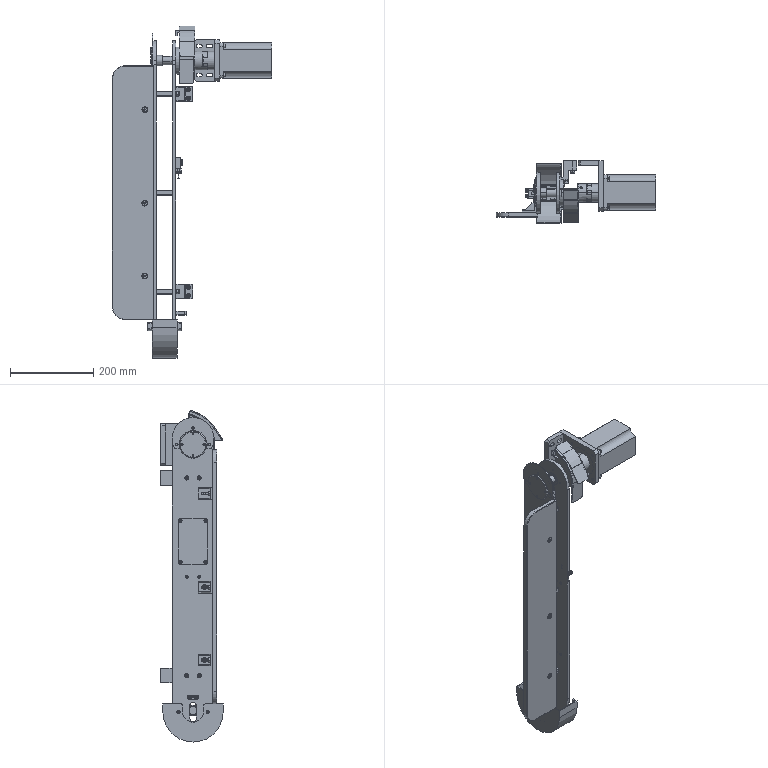Assembly | SolidWorks | mm | 101 component files | 105 solids | 2429 faces | box 382.9 x 150 x 797.7 mm | volume 3111825 mm3 | plane 1200 | cylinder 794 | cone 339 | torus 80 | sphere 12 | spline 4 | commonest cylinder face diameters 6 x114 6.68 x66 9.88 x66 5 x64 4 x49 10 x49 8.5 x32 7 x28
Bill of materials:
Deep Groove Ball Bearing, Double Sealed, 6804ZZ | 2 | 304 Stainless Steel | Flat annular ring (washer- or spacer-like): short cylinder with a large concentric through bore.
A3 Steel | 1 | A3 Steel | Thick circular flange disc with a central through bore and four small through holes evenly spaced on a bolt circle.
A3 Steel | 1 | A3 Steel | Thin circular plate with four small through holes evenly spaced on a bolt circle and no central through hole.
A3 Steel | 1 | 40Cr | Short cylindrical shaft or pin with a raised central collar and flats machined on both end sections.
A3 Steel | 2 | A3 Steel | Rectangular block with one through hole in the top face and two parallel through holes crossing it horizontally; the four vertical edges are chamfered.
Stainless Steel304 | 1 | 40Cr | Thin-walled cylindrical sleeve or bushing with chamfered edges at both ends.
A3 Steel | 1 | 40Cr | Stepped cylindrical shaft with a narrow raised ring partway along it, a reduced-diameter end journal and a keyway-like slot at the small end.
Stainless Steel304 | 1 | 40Cr | Cylindrical sleeve or bushing, longer than unnamed part, with chamfered edges at both ends.
A3 Steel | 1 | 201 Stainless Steel | Thin flat horseshoe- or C-shaped plate (partial annulus) with three small through holes: one at the crown and one near each end of the arms.
A3 Steel | 1 | A3 Steel | Long thin flat strip with fully rounded ends, a round hole at one end, an elongated slot at the other end, and several groups of very small holes along its length.
A3 Steel | 3 | A3 Steel | Rectangular block with chamfered vertical edges and two blind drilled holes on one face that end in conical drill points.
A3 Steel | 1 | A3 Steel | Rectangular flat mounting-style plate with one large circular through opening, six small through holes and two chamfered corners on one side.
A3 Steel | 1 | A3 Steel | Rectangular block-like plate with four obround through-slots in the main face, two chamfered corners on one long edge, and two small holes in one narrow side face.
A3 Steel | 1 | A3 Steel | Long, thin flat plate with rounded ends. It has a round hole near one end, an obround slot near the other end, a rectangular window toward the upper middle, and many small holes in a pattern.
A3 Steel | 1 | A3 Steel | Stepped rectangular block: a taller, narrower upper column sits on a wider, shorter base. A long obround slot passes through the column's narrow side, and the base has two round through-holes.
Stainless Steel201 | 1 | 201 Stainless Steel | Half-cylindrical, trough- or cradle-like shell with thin curved walls. One end has a flat semicircular end face with a central U-shaped cutout and two small holes, one in each flat upper tab.
A3 Steel | 2 | A3 Steel | Block with a Z-shaped, stepped profile made of two offset rectangular lobes with filleted inside corners. One face has two large through-holes; another face has three holes in a row, with the middle one smaller. The outer corners have small chamfers.
Bakelite Red | 1 | Bakelite (Red) | Long, thin flat strip with two rounded corners on one long edge and three small holes evenly spaced near the opposite edge. A small step shows at one end in the edge view.
Stainless Steel201 | 1 | 201 Stainless Steel | Bent, sheet-like bracket with a curved, angled upper flange and a flat lower tab. The flat profile has two obround slots and an irregular outline with filleted notches. A small hooked tab sticks out to one side.
Acrylic PMMA Transparent | 1 | PMMA Transparent | Thin rectangular flat plate with rounded corners and one small round hole near each of the four corners.
Coupling075-12.7-14 | 1 |  | Solid cylinder with chamfered ends and a central axial bore that appears to have a keyway. Several partial circumferential slits, offset around the circumference, cut through the body, and there is one radial hole near one end.
Foot | 3 |  | Right-angle corner bracket with two perpendicular legs joined by a solid diagonal (gusset-like) web. Each leg has one obround slot, and the leg ends have rounded corners.
GB_FASTENER_NUT_SNAB1 M6-N | 3 |  | Hexagonal nut-like prism with a plain round through-bore and chamfered corners on both faces
hex socket set screws with flat point gb | 2 |  | Short cylinder with a hexagonal socket recess in one end face and a conical, pointed or chamfered tip at the other end. There is a small chamfer at the socket end.
GB_SOCKET_TYPE7 M4X10-N | 6 |  | Pin with a domed head and a plain cylindrical shank with a flat end, like a round-head rivet or pin
GB_FASTENER_SCREWS_HSCHS M6X16-N | 3 |  | Countersunk (conical underside) flat-head fastener with a hexagonal socket recess and a plain cylindrical shank with a chamfered tip
Socket Head Cap Screw M3X20 | 2 |  | Long, slender socket-head cap-screw-like part: a cylindrical head with a hex socket and a long plain shank
GB_FASTENER_SCREWS_HSHCS M6X16-N | 16 |  | Short socket-head cap-screw-like part: a cylindrical head with a hex socket and a short, thicker plain shank
GB_FASTENER_SCREWS_HSHCS M5X25-C | 4 |  | Cylindrical-head pin or screw-like part with a long plain shank; the head's top face is not visible
GB_FASTENER_SCREWS_HSHCS M5X20-N | 4 |  | Socket-head cap-screw-like part: a cylindrical head with a hex socket and a plain cylindrical shank of medium length
GB_FASTENER_SCREWS_HSHCS M5X12-N | 2 |  | Short cylindrical-head pin or screw-like part with a thick plain shank; the head's top face is not visible
M3 Flat Washer | 2 |  | Thin flat annular washer-like disc with a central round hole
GB_FASTENER_WASHER_SMWC 6 | 2 |  | Flat annular ring/washer-like part, thicker than the thin washer, with a relatively large central hole
SlotTypeProximitySwitchEE-SX951-W | 1 |  | U-shaped, forked rectangular block with a rectangular slot between two arms. One face has two round holes, a cylindrical rod or stub sticks out from the underside, and there are small line marks on the top surface.
M4 Spring Washer | 2 |  | Split ring with a single radial cut and slightly offset ends, like a split lock washer
GB_FASTENER_WASHER_SW 6 | 14 |  | Split ring with a single radial cut and slightly offset ends, like a split lock washer; it looks nearly identical to unnamed part
M6 Spring Washer | 8 |  | Flat annular ring with a rectangular cross-section, cut through by one narrow radial split. The two cut ends look slightly offset along the axis, which fits a split (helical) lock-washer-style shape.
StepperMotor86J18118-842 | 1 |  | Elongated square-section prismatic body with concave, quarter-round reliefs running the full length of each longitudinal corner. One end has a slightly larger square flange with rounded corners and four corner through-holes, a thin raised circular boss (pilot) on its outer face, and a single plain cylindrical shaft sticking out along the central axis. The overall form looks like a compact motor-style housing with a mounting flange and output shaft.
Mates:
1. coincident | ChainPartSupport-1 face at (155.637, 19.937, -132.704) dir (1, 0, 0) | ChainPartSupport-2 face at (155.637, 19.937, -607.704) dir (1, 0, 0)
2. concentric | ChainPartInnerSidePlate-1 face at (127.637, -2.563, -35.304) dir (1, 0, 0) r 16 | ChainPartOuterSidePlate-1 face at (88.237, -2.563, -35.304) dir (-1, 0, 0) r 16
3. concentric | ChainPartInnerSidePlate-1 face at (127.637, -2.563, -670.304) dir (1, 0, 0) r 48.5 | ChainPartOuterSidePlate-1 face at (88.237, -2.563, -670.304) dir (-1, 0, 0) r 48.5
4. coincident | ChainPartInnerSidePlate-1 face at (127.637, -2.563, -35.304) dir (-1, 0, 0) | ChainPartInnerSpacer-1 face at (127.637, -2.563, -115.304) dir (1, 0, 0)
5. concentric | ChainPartInnerSidePlate-1 face at (137.637, 12.437, -115.304) dir (-1, 0, 0) r 3.5 | ChainPartInnerSpacer-1 face at (88.237, 12.437, -115.304) dir (-1, 0, 0) r 3
6. concentric | ChainPartInnerSidePlate-1 face at (137.637, -17.563, -115.304) dir (-1, 0, 0) r 3.5 | ChainPartInnerSpacer-1 face at (88.237, -17.563, -115.304) dir (-1, 0, 0) r 3
7. coincident | ChainPartOuterSidePlate-1 face at (88.237, -2.563, -35.304) dir (1, 0, 0) | ChainPartInnerSpacer-1 face at (88.237, -2.563, -115.304) dir (-1, 0, 0)
8. concentric | ChainPartInnerSidePlate-1 face at (137.637, 12.437, -590.304) dir (-1, 0, 0) r 3.5 | ChainPartInnerSpacer-3 face at (88.237, 12.437, -590.304) dir (-1, 0, 0) r 3
9. concentric | ChainPartInnerSidePlate-1 face at (127.637, -2.563, -35.304) dir (1, 0, 0) r 16 | Bearing_6804ZZ-1 face at (135.637, -2.563, -35.304) dir (-1, 0, 0) r 16
10. concentric | ChainPartDriveShaft-1 face at (198.637, -2.563, -35.304) dir (1, 0, 0) r 10 | Bearing_6804ZZ-1 face at (135.637, -2.563, -35.304) dir (-1, 0, 0) r 10
11. coincident | ChainPartDriveShaft-1 face at (128.637, -0.9828, -45.178) dir (1, 0, 0) | Bearing_6804ZZ-1 face at (128.637, 8.267, -39.461) dir (-1, 0, 0)
12. concentric | ChainPartDriveShaft-1 face at (198.637, -2.563, -35.304) dir (1, 0, 0) r 10 | Bearing_6804ZZ-2 face at (87.237, -2.563, -35.304) dir (-1, 0, 0) r 10
13. coincident | ChainPartOuterSidePlate-1 face at (80.237, -2.563, -35.304) dir (-1, 0, 0) | Bearing_6804ZZ-2 face at (80.237, 12.094, -40.931) dir (-1, 0, 0)
14. coincident | ChainPartInnerSidePlate-1 face at (135.637, -2.563, -35.304) dir (1, 0, 0) | Bearing_6804ZZ-1 face at (135.637, 11.086, -40.544) dir (1, 0, 0)
15. coincident | ChainPartInnerSidePlate-1 face at (127.637, -2.563, -35.304) dir (-1, 0, 0) | ChainPartDrivenShaft-1 face at (127.637, -15.063, -673.885) dir (1, 0, 0)
16. coincident | ChainPartInnerSidePlate-1 face at (125.637, 5.437, -662.304) dir (0, -1, 0) | ChainPartDrivenShaft-1 face at (127.637, 5.437, -693.885) dir (0, 1, 0)
17. coincident | ChainPartInnerSidePlate-1 face at (135.637, -2.563, -35.304) dir (1, 0, 0) | ChainPartBearingInnerEndCap-1 face at (135.637, 29.937, -35.304) dir (-1, 0, 0)
18. concentric | ChainPartDriveShaft-1 face at (198.637, -2.563, -35.304) dir (1, 0, 0) r 10 | ChainPartBearingInnerEndCap-1 face at (145.437, -2.563, -35.304) dir (1, 0, 0) r 10.5
19. concentric | ChainPartInnerSidePlate-1 face at (127.637, -2.563, -9.304) dir (-1, 0, 0) r 1.65 | ChainPartBearingInnerEndCap-1 face at (145.437, -2.563, -9.304) dir (1, 0, 0) r 2.25
20. coincident | ChainPartOuterSidePlate-1 face at (80.237, -2.563, -35.304) dir (-1, 0, 0) | ChainPartBearingOuterEndCap-1 face at (80.237, -35.063, -35.304) dir (1, 0, 0)
21. concentric | ChainPartOuterSidePlate-1 face at (80.737, -2.563, -35.304) dir (1, 0, 0) r 785.398 | ChainPartBearingOuterEndCap-1 face at (75.437, -2.563, -35.304) dir (-1, 0, 0) r 32.5
22. concentric | ChainPartOuterSidePlate-1 face at (88.237, 23.437, -35.304) dir (1, 0, 0) r 2 | ChainPartBearingOuterEndCap-1 face at (75.437, 23.437, -35.304) dir (-1, 0, 0) r 2.25
23. coincident | Bearing_6804ZZ-2 face at (87.237, 11.086, -40.544) dir (1, 0, 0) | ChainPartDriveShaftLocatingSleeve-1 face at (87.237, -2.563, -35.304) dir (-1, 0, 0)
24. concentric | ChainPartDriveShaft-1 face at (198.637, -2.563, -35.304) dir (1, 0, 0) r 10 | ChainPartDriveShaftLocatingSleeve-1 face at (104.337, -2.563, -35.304) dir (-1, 0, 0) r 12.5
25. coincident | ChainPartOuterSidePlate-1 face at (88.237, -2.563, -35.304) dir (1, 0, 0) | ChainPartDrivenShaftLocatingSleeve-1 face at (88.237, -2.563, -673.885) dir (-1, 0, 0)
26. concentric | ChainPartDrivenShaft-1 face at (67.237, -2.563, -673.885) dir (-1, 0, 0) r 10 | ChainPartDrivenShaftLocatingSleeve-1 face at (100.937, -2.563, -673.885) dir (-1, 0, 0) r 12.5
27. coincident | ChainPartOuterSidePlate-1 face at (80.237, -2.563, -35.304) dir (-1, 0, 0) | ChainPartWindowPlate-1 face at (80.237, -32.563, -317.804) dir (1, 0, 0)
28. concentric | ChainPartOuterSidePlate-1 face at (80.237, 27.437, -217.804) dir (-1, 0, 0) r 2 | ChainPartWindowPlate-1 face at (77.237, 27.437, -217.804) dir (1, 0, 0) r 2.25
29. concentric | ChainPartOuterSidePlate-1 face at (80.237, 27.437, -317.804) dir (-1, 0, 0) r 2 | ChainPartWindowPlate-1 face at (77.237, 27.437, -317.804) dir (1, 0, 0) r 2.25
30. concentric | ChainPartInnerSidePlate-1 face at (135.637, 4.437, -642.304) dir (1, 0, 0) r 2.5 | ChainPartDrivenShaftAdjustmentBracket-2 face at (135.637, 4.437, -642.304) dir (1, 0, 0) r 2.75
31. concentric | ChainPartInnerSidePlate-1 face at (135.637, -9.563, -642.304) dir (1, 0, 0) r 2.5 | ChainPartDrivenShaftAdjustmentBracket-2 face at (135.637, -9.563, -642.304) dir (1, 0, 0) r 2.75
32. concentric | ChainPartOuterSidePlate-1 face at (80.237, 4.437, -642.304) dir (-1, 0, 0) r 2.5 | ChainPartDrivenShaftAdjustmentBracket-4 face at (80.237, 4.437, -642.304) dir (-1, 0, 0) r 2.75
33. concentric | ChainPartOuterSidePlate-1 face at (80.237, -9.563, -642.304) dir (-1, 0, 0) r 2.5 | ChainPartDrivenShaftAdjustmentBracket-4 face at (80.237, -9.563, -642.304) dir (-1, 0, 0) r 2.75
34. concentric | ChainPartSupport-1 face at (155.637, 27.437, -125.304) dir (1, 0, 0) r 5.5 | ChainPartInnerSidePlate-1 face at (127.637, 27.437, -125.304) dir (-1, 0, 0) r 3
35. concentric | ChainPartSupport-1 face at (155.637, 27.437, -105.304) dir (1, 0, 0) r 5.5 | ChainPartInnerSidePlate-1 face at (127.637, 27.437, -105.304) dir (-1, 0, 0) r 3
36. concentric | ChainPartSupport-2 face at (155.637, 27.437, -580.304) dir (1, 0, 0) r 5.5 | ChainPartInnerSidePlate-1 face at (127.637, 27.437, -580.304) dir (-1, 0, 0) r 3
37. concentric | ChainPartSupport-2 face at (155.637, 27.437, -600.304) dir (1, 0, 0) r 5.5 | ChainPartInnerSidePlate-1 face at (127.637, 27.437, -600.304) dir (-1, 0, 0) r 3
38. concentric | ChainPartDriveShaft-1 face at (198.637, -2.563, -35.304) dir (1, 0, 0) r 7 | Coupling075-12.7-14-1 face at (199.337, -2.563, -35.304) dir (-1, 0, 0) r 7
39. coincident | ChainPartDriveShaft-1 face at (178.637, -1.457, -42.216) dir (1, 0, 0) | Coupling075-12.7-14-1 face at (178.637, -22.592, -12.658) dir (-1, 0, 0)
40. concentric | Coupling075-12.7-14-1 face at (178.636, -2.563, -35.304) dir (1, 0, 0) r 6.35 | StepperMotor86J18118-842-1 face at (209.117, -2.563, -35.304) dir (1, 0, 0) r 6.35
41. distance | StepperMotor86J18118-842-1 face at (239.117, -2.563, -35.304) dir (-1, 0, 0) | Coupling075-12.7-14-1 face at (232.737, 19.843, -15.006) dir (1, 0, 0)
42. coincident | ChainPartOuterSidePlate-1 face at (80.237, -52.063, -35.304) dir (0, -1, 0) | ChainPartTablePlate-1 face at (32.737, -52.063, -352.804) dir (0, 1, 0)
43. coincident | ChainPartOuterSidePlate-1 face at (80.237, -2.563, -35.304) dir (-1, 0, 0) | ChainPartTablePlate-1 face at (80.237, -52.063, -657.804) dir (1, 0, 0)
44. coincident | ChainPartSupport-1 face at (135.637, 74.937, -132.704) dir (-1, 0, 0) | ChainPartInnerSidePlate-1 face at (135.637, -2.563, -35.304) dir (1, 0, 0)
45. coincident | ChainPartTablePlate-1 face at (-17.263, -50.063, -657.804) dir (0, 1, 0) | Foot-1 face at (80.237, -50.063, -138.804) dir (0, -1, 0)
46. coincident | ChainPartOuterSidePlate-1 face at (80.237, -2.563, -35.304) dir (-1, 0, 0) | Foot-1 face at (80.237, -50.063, -138.804) dir (1, 0, 0)
47. coincident | ChainPartOuterSidePlate-1 face at (80.237, -2.563, -35.304) dir (-1, 0, 0) | Foot-2 face at (80.237, -50.063, -538.804) dir (1, 0, 0)
48. concentric | ChainPartOuterSidePlate-1 face at (80.237, -30.563, -552.804) dir (-1, 0, 0) r 2.5 | Foot-2 sketch point at (75.637, -30.563, -552.804) dir (1, 0, 0)
49. coincident | ChainPartOuterSidePlate-1 face at (88.237, -2.563, -35.304) dir (1, 0, 0) | ChainPartInnerSpacer-3 face at (88.237, -2.563, -590.304) dir (-1, 0, 0)
50. concentric | ChainPartBearingInnerEndCap-1 face at (145.437, -28.563, -35.304) dir (1, 0, 0) r 2.25 | ChainPartThreadGuide-1 sketch point at (160.737, -28.563, -35.304) dir (1, 0, 0)
51. coincident | ChainPartOuterSidePlate-1 face at (80.237, -2.563, -35.304) dir (-1, 0, 0) | ChainPartDrivenShaftAdjustmentBracket-4 face at (80.237, -2.563, -642.304) dir (1, 0, 0)
52. coincident | ChainPartInnerSidePlate-1 face at (135.637, -2.563, -35.304) dir (1, 0, 0) | ChainPartDrivenShaftAdjustmentBracket-2 face at (135.637, -2.563, -642.304) dir (-1, 0, 0)
53. concentric | StepperMotor86J18118-842-1 face at (365.637, -37.313, -0.5537) dir (-1, 0, 0) r 2.75 | spring lock washers--normal type gb-30 face at (249.137, -37.313, -0.5537) dir (1, 0, 0) r 3.34
54. coincident | StepperMotor86J18118-842-1 face at (249.137, -44.384, 6.517) dir (1, 0, 0) | spring lock washers--normal type gb-30 face at (249.137, -37.313, -0.5537) dir (-1, 0, 0)
55. concentric | StepperMotor86J18118-842-1 face at (365.637, -37.313, -70.054) dir (-1, 0, 0) r 2.75 | spring lock washers--normal type gb-31 face at (249.137, -37.313, -70.054) dir (1, 0, 0) r 3.34
56. coincident | StepperMotor86J18118-842-1 face at (249.137, -44.384, -77.125) dir (1, 0, 0) | spring lock washers--normal type gb-31 face at (249.137, -37.313, -70.054) dir (-1, 0, 0)
57. concentric | StepperMotor86J18118-842-1 face at (365.637, 32.187, -0.5537) dir (-1, 0, 0) r 2.75 | spring lock washers--normal type gb-28 face at (249.137, 32.187, -0.5537) dir (1, 0, 0) r 3.34
58. coincident | StepperMotor86J18118-842-1 face at (249.137, 39.258, 6.517) dir (1, 0, 0) | spring lock washers--normal type gb-28 face at (249.137, 32.187, -0.5537) dir (-1, 0, 0)
59. concentric | StepperMotor86J18118-842-1 edge at (249.137, 32.187, -70.054) dir (1, 0, 0) r 2.75 | spring lock washers--normal type gb-29 face at (249.137, 32.187, -70.054) dir (1, 0, 0) r 3.34
60. coincident | StepperMotor86J18118-842-1 face at (249.137, 39.258, -77.125) dir (1, 0, 0) | spring lock washers--normal type gb-29 face at (249.137, 32.187, -70.054) dir (-1, 0, 0)
61. concentric | StepperMotor86J18118-842-1 face at (365.637, -37.313, -0.5537) dir (-1, 0, 0) r 2.75 | hexagon socket head cap screws gb-29 face at (230.737, -37.313, -0.5537) dir (1, 0, 0) r 2.5
62. coincident | spring lock washers--normal type gb-30 face at (250.737, -37.313, -0.5537) dir (1, 0, 0) | hexagon socket head cap screws gb-29 face at (250.737, -37.313, -0.5537) dir (-1, 0, 0)
63. concentric | spring lock washers--normal type gb-31 face at (249.137, -37.313, -70.054) dir (1, 0, 0) r 3.34 | hexagon socket head cap screws gb-30 face at (230.737, -37.313, -70.054) dir (1, 0, 0) r 2.5
64. coincident | spring lock washers--normal type gb-31 face at (250.737, -37.313, -70.054) dir (1, 0, 0) | hexagon socket head cap screws gb-30 face at (250.737, -37.313, -70.054) dir (-1, 0, 0)
65. concentric | spring lock washers--normal type gb-28 face at (249.137, 32.187, -0.5537) dir (1, 0, 0) r 3.34 | hexagon socket head cap screws gb-31 face at (230.737, 32.187, -0.5537) dir (1, 0, 0) r 2.5
66. coincident | spring lock washers--normal type gb-28 face at (250.737, 32.187, -0.5537) dir (1, 0, 0) | hexagon socket head cap screws gb-31 face at (250.737, 32.187, -0.5537) dir (-1, 0, 0)
67. concentric | spring lock washers--normal type gb-29 face at (249.137, 32.187, -70.054) dir (1, 0, 0) r 3.34 | hexagon socket head cap screws gb-32 face at (230.737, 32.187, -70.054) dir (1, 0, 0) r 2.5
68. coincident | spring lock washers--normal type gb-29 face at (250.737, 32.187, -70.054) dir (1, 0, 0) | hexagon socket head cap screws gb-32 face at (250.737, 32.187, -70.054) dir (-1, 0, 0)
69. coincident | ChainPartOuterSidePlate-1 face at (80.237, -2.563, -35.304) dir (-1, 0, 0) | ChainPartRearCover-1 face at (80.237, -2.563, -677.304) dir (1, 0, 0)
70. concentric | ChainPartOuterSidePlate-1 face at (80.237, -37.563, -677.304) dir (-1, 0, 0) r 2.5 | ChainPartRearCover-1 face at (88.237, -37.563, -677.304) dir (-1, 0, 0) r 3
71. concentric | ChainPartOuterSidePlate-1 face at (80.237, 32.437, -677.304) dir (-1, 0, 0) r 2.5 | ChainPartRearCover-1 face at (88.237, 32.437, -677.304) dir (-1, 0, 0) r 3
72. concentric | ChainPartRearCover-1 face at (88.237, -37.563, -677.304) dir (-1, 0, 0) r 3 | hexagon socket button head screws gb-4 face at (88.237, -37.563, -677.304) dir (-1, 0, 0) r 2
73. coincident | ChainPartRearCover-1 face at (78.237, -2.563, -677.304) dir (-1, 0, 0) | hexagon socket button head screws gb-4 face at (78.237, -37.563, -677.304) dir (1, 0, 0)
74. concentric | ChainPartRearCover-1 face at (88.237, 32.437, -677.304) dir (-1, 0, 0) r 3 | hexagon socket button head screws gb-5 face at (88.237, 32.437, -677.304) dir (-1, 0, 0) r 2
75. coincident | ChainPartRearCover-1 face at (78.237, -2.563, -677.304) dir (-1, 0, 0) | hexagon socket button head screws gb-5 face at (78.237, 32.437, -677.304) dir (1, 0, 0)
76. concentric | ChainPartWindowPlate-1 face at (77.237, 27.437, -317.804) dir (1, 0, 0) r 2.25 | hexagon socket button head screws gb-6 face at (87.237, 27.437, -317.804) dir (-1, 0, 0) r 2
77. coincident | ChainPartWindowPlate-1 face at (77.237, -32.563, -317.804) dir (-1, 0, 0) | hexagon socket button head screws gb-6 face at (77.237, 27.437, -317.804) dir (1, 0, 0)
78. concentric | ChainPartWindowPlate-1 face at (77.237, -32.563, -317.804) dir (1, 0, 0) r 2.25 | hexagon socket button head screws gb-7 face at (87.237, -32.563, -317.804) dir (-1, 0, 0) r 2
79. coincident | ChainPartWindowPlate-1 face at (77.237, -32.563, -317.804) dir (-1, 0, 0) | hexagon socket button head screws gb-7 face at (77.237, -32.563, -317.804) dir (1, 0, 0)
80. concentric | ChainPartWindowPlate-1 face at (77.237, -32.563, -217.804) dir (1, 0, 0) r 2.25 | hexagon socket button head screws gb-8 face at (87.237, -32.563, -217.804) dir (-1, 0, 0) r 2
81. coincident | ChainPartWindowPlate-1 face at (77.237, -32.563, -317.804) dir (-1, 0, 0) | hexagon socket button head screws gb-8 face at (77.237, -32.563, -217.804) dir (1, 0, 0)
82. concentric | ChainPartWindowPlate-1 face at (77.237, 27.437, -217.804) dir (1, 0, 0) r 2.25 | hexagon socket button head screws gb-9 face at (87.237, 27.437, -217.804) dir (-1, 0, 0) r 2
83. coincident | ChainPartWindowPlate-1 face at (77.237, -32.563, -317.804) dir (-1, 0, 0) | hexagon socket button head screws gb-9 face at (77.237, 27.437, -217.804) dir (1, 0, 0)
84. concentric | ChainPartInnerSidePlate-1 face at (137.637, -17.563, -590.304) dir (-1, 0, 0) r 3.5 | ChainPartInnerSpacer-3 face at (88.237, -17.563, -590.304) dir (-1, 0, 0) r 3
85. concentric | ChainPartOuterSidePlate-1 face at (78.237, -17.563, -115.304) dir (1, 0, 0) r 3.5 | spring lock washers--normal type gb-16 face at (80.237, -17.563, -115.304) dir (-1, 0, 0) r 3.34
86. coincident | ChainPartOuterSidePlate-1 face at (80.237, -2.563, -35.304) dir (-1, 0, 0) | spring lock washers--normal type gb-16 face at (80.237, -17.563, -115.304) dir (1, 0, 0)
87. concentric | ChainPartOuterSidePlate-1 face at (78.237, 12.437, -115.304) dir (1, 0, 0) r 3.5 | spring lock washers--normal type gb-17 face at (80.237, 12.437, -115.304) dir (-1, 0, 0) r 3.34
88. coincident | ChainPartOuterSidePlate-1 face at (80.237, -2.563, -35.304) dir (-1, 0, 0) | spring lock washers--normal type gb-17 face at (80.237, 12.437, -115.304) dir (1, 0, 0)
89. concentric | ChainPartOuterSidePlate-1 face at (78.237, -17.563, -590.304) dir (1, 0, 0) r 3.5 | spring lock washers--normal type gb-18 face at (80.237, -17.563, -590.304) dir (-1, 0, 0) r 3.34
90. coincident | ChainPartOuterSidePlate-1 face at (80.237, -2.563, -35.304) dir (-1, 0, 0) | spring lock washers--normal type gb-18 face at (80.237, -17.563, -590.304) dir (1, 0, 0)
91. concentric | ChainPartOuterSidePlate-1 face at (78.237, 12.437, -590.304) dir (1, 0, 0) r 3.5 | spring lock washers--normal type gb-19 face at (80.237, 12.437, -590.304) dir (-1, 0, 0) r 3.34
92. coincident | ChainPartOuterSidePlate-1 face at (80.237, -2.563, -35.304) dir (-1, 0, 0) | spring lock washers--normal type gb-19 face at (80.237, 12.437, -590.304) dir (1, 0, 0)
93. concentric | ChainPartInnerSidePlate-1 face at (137.637, -17.563, -115.304) dir (-1, 0, 0) r 3.5 | spring lock washers--normal type gb-20 face at (135.637, -17.563, -115.304) dir (1, 0, 0) r 3.34
94. coincident | ChainPartInnerSidePlate-1 face at (135.637, -2.563, -35.304) dir (1, 0, 0) | spring lock washers--normal type gb-20 face at (135.637, -17.563, -115.304) dir (-1, 0, 0)
95. concentric | ChainPartInnerSidePlate-1 face at (137.637, 12.437, -115.304) dir (-1, 0, 0) r 3.5 | spring lock washers--normal type gb-21 face at (135.637, 12.437, -115.304) dir (1, 0, 0) r 3.34
96. coincident | ChainPartInnerSidePlate-1 face at (135.637, -2.563, -35.304) dir (1, 0, 0) | spring lock washers--normal type gb-21 face at (135.637, 12.437, -115.304) dir (-1, 0, 0)
97. concentric | ChainPartInnerSidePlate-1 face at (137.637, -17.563, -590.304) dir (-1, 0, 0) r 3.5 | spring lock washers--normal type gb-22 face at (135.637, -17.563, -590.304) dir (1, 0, 0) r 3.34
98. coincident | ChainPartInnerSidePlate-1 face at (135.637, -2.563, -35.304) dir (1, 0, 0) | spring lock washers--normal type gb-22 face at (135.637, -17.563, -590.304) dir (-1, 0, 0)
99. concentric | ChainPartInnerSidePlate-1 face at (137.637, 12.437, -590.304) dir (-1, 0, 0) r 3.5 | spring lock washers--normal type gb-23 face at (135.637, 12.437, -590.304) dir (1, 0, 0) r 3.34
100. coincident | ChainPartInnerSidePlate-1 face at (135.637, -2.563, -35.304) dir (1, 0, 0) | spring lock washers--normal type gb-23 face at (135.637, 12.437, -590.304) dir (-1, 0, 0)
101. concentric | spring lock washers--normal type gb-19 face at (80.237, 12.437, -590.304) dir (-1, 0, 0) r 4.94 | hexagon socket head cap screws gb-17 face at (94.637, 12.437, -590.304) dir (-1, 0, 0) r 3
102. coincident | spring lock washers--normal type gb-19 face at (78.637, 12.437, -590.304) dir (-1, 0, 0) | hexagon socket head cap screws gb-17 face at (78.637, 12.437, -590.304) dir (1, 0, 0)
103. concentric | spring lock washers--normal type gb-18 face at (80.237, -17.563, -590.304) dir (-1, 0, 0) r 3.34 | hexagon socket head cap screws gb-18 face at (94.637, -17.563, -590.304) dir (-1, 0, 0) r 3
104. coincident | spring lock washers--normal type gb-18 face at (78.637, -17.563, -590.304) dir (-1, 0, 0) | hexagon socket head cap screws gb-18 face at (78.637, -17.563, -590.304) dir (1, 0, 0)
105. concentric | spring lock washers--normal type gb-16 face at (80.237, -17.563, -115.304) dir (-1, 0, 0) r 3.34 | hexagon socket head cap screws gb-19 face at (94.637, -17.563, -115.304) dir (-1, 0, 0) r 3
106. coincident | spring lock washers--normal type gb-16 face at (78.637, -17.563, -115.304) dir (-1, 0, 0) | hexagon socket head cap screws gb-19 face at (78.637, -17.563, -115.304) dir (1, 0, 0)
107. concentric | spring lock washers--normal type gb-17 face at (80.237, 12.437, -115.304) dir (-1, 0, 0) r 3.34 | hexagon socket head cap screws gb-20 face at (94.637, 12.437, -115.304) dir (-1, 0, 0) r 3
108. coincident | spring lock washers--normal type gb-17 face at (78.637, 12.437, -115.304) dir (-1, 0, 0) | hexagon socket head cap screws gb-20 face at (78.637, 12.437, -115.304) dir (1, 0, 0)
109. concentric | spring lock washers--normal type gb-20 face at (135.637, -17.563, -115.304) dir (1, 0, 0) r 3.34 | hexagon socket head cap screws gb-21 face at (121.237, -17.563, -115.304) dir (1, 0, 0) r 3
110. coincident | spring lock washers--normal type gb-20 face at (137.237, -17.563, -115.304) dir (1, 0, 0) | hexagon socket head cap screws gb-21 face at (137.237, -17.563, -115.304) dir (-1, 0, 0)
111. concentric | spring lock washers--normal type gb-21 face at (135.637, 12.437, -115.304) dir (1, 0, 0) r 3.34 | hexagon socket head cap screws gb-22 face at (121.237, 12.437, -115.304) dir (1, 0, 0) r 3
112. coincident | spring lock washers--normal type gb-21 face at (137.237, 12.437, -115.304) dir (1, 0, 0) | hexagon socket head cap screws gb-22 face at (137.237, 12.437, -115.304) dir (-1, 0, 0)
113. concentric | spring lock washers--normal type gb-22 face at (135.637, -17.563, -590.304) dir (1, 0, 0) r 3.34 | hexagon socket head cap screws gb-23 face at (121.237, -17.563, -590.304) dir (1, 0, 0) r 3
114. coincident | spring lock washers--normal type gb-22 face at (137.237, -17.563, -590.304) dir (1, 0, 0) | hexagon socket head cap screws gb-23 face at (137.237, -17.563, -590.304) dir (-1, 0, 0)
115. concentric | spring lock washers--normal type gb-23 face at (135.637, 12.437, -590.304) dir (1, 0, 0) r 3.34 | hexagon socket head cap screws gb-24 face at (121.237, 12.437, -590.304) dir (1, 0, 0) r 3
116. coincident | spring lock washers--normal type gb-23 face at (137.237, 12.437, -590.304) dir (1, 0, 0) | hexagon socket head cap screws gb-24 face at (137.237, 12.437, -590.304) dir (-1, 0, 0)
117. concentric | ChainPartDrivenShaftAdjustmentBracket-4 face at (80.237, -9.563, -642.304) dir (-1, 0, 0) r 2.75 | spring lock washers--normal type gb-24 face at (60.437, -9.563, -642.304) dir (-1, 0, 0) r 3.34
118. coincident | ChainPartDrivenShaftAdjustmentBracket-4 face at (60.437, -2.563, -642.304) dir (-1, 0, 0) | spring lock washers--normal type gb-24 face at (60.437, -9.563, -642.304) dir (1, 0, 0)
119. concentric | ChainPartDrivenShaftAdjustmentBracket-4 face at (80.237, 4.437, -642.304) dir (-1, 0, 0) r 2.75 | spring lock washers--normal type gb-25 face at (60.437, 4.437, -642.304) dir (-1, 0, 0) r 3.34
120. coincident | ChainPartDrivenShaftAdjustmentBracket-4 face at (60.437, -2.563, -642.304) dir (-1, 0, 0) | spring lock washers--normal type gb-25 face at (60.437, 4.437, -642.304) dir (1, 0, 0)
121. concentric | ChainPartDrivenShaftAdjustmentBracket-2 face at (135.637, -9.563, -642.304) dir (1, 0, 0) r 2.75 | spring lock washers--normal type gb-26 face at (155.437, -9.563, -642.304) dir (1, 0, 0) r 3.34
122. coincident | ChainPartDrivenShaftAdjustmentBracket-2 face at (155.437, -2.563, -642.304) dir (1, 0, 0) | spring lock washers--normal type gb-26 face at (155.437, -9.563, -642.304) dir (-1, 0, 0)
123. concentric | ChainPartDrivenShaftAdjustmentBracket-2 face at (135.637, 4.437, -642.304) dir (1, 0, 0) r 2.75 | spring lock washers--normal type gb-27 face at (155.437, 4.437, -642.304) dir (1, 0, 0) r 3.34
124. coincident | ChainPartDrivenShaftAdjustmentBracket-2 face at (155.437, -2.563, -642.304) dir (1, 0, 0) | spring lock washers--normal type gb-27 face at (155.437, 4.437, -642.304) dir (-1, 0, 0)
125. concentric | ChainPartDrivenShaftAdjustmentBracket-4 face at (80.237, -9.563, -642.304) dir (-1, 0, 0) r 2.75 | hexagon socket head cap screws gb-25 face at (83.837, -9.563, -642.304) dir (-1, 0, 0) r 2.5
126. coincident | spring lock washers--normal type gb-24 face at (58.837, -9.563, -642.304) dir (-1, 0, 0) | hexagon socket head cap screws gb-25 face at (58.837, -9.563, -642.304) dir (1, 0, 0)
127. concentric | spring lock washers--normal type gb-25 face at (60.437, 4.437, -642.304) dir (-1, 0, 0) r 3.34 | hexagon socket head cap screws gb-26 face at (83.837, 4.437, -642.304) dir (-1, 0, 0) r 2.5
128. coincident | spring lock washers--normal type gb-25 face at (58.837, 4.437, -642.304) dir (-1, 0, 0) | hexagon socket head cap screws gb-26 face at (58.837, 4.437, -642.304) dir (1, 0, 0)
129. concentric | spring lock washers--normal type gb-26 face at (155.437, -9.563, -642.304) dir (1, 0, 0) r 3.34 | hexagon socket head cap screws gb-27 face at (132.037, -9.563, -642.304) dir (1, 0, 0) r 2.5
130. coincident | spring lock washers--normal type gb-26 face at (157.037, -9.563, -642.304) dir (1, 0, 0) | hexagon socket head cap screws gb-27 face at (157.037, -9.563, -642.304) dir (-1, 0, 0)
131. concentric | spring lock washers--normal type gb-27 face at (155.437, 4.437, -642.304) dir (1, 0, 0) r 3.34 | hexagon socket head cap screws gb-28 face at (132.037, 4.437, -642.304) dir (1, 0, 0) r 2.5
132. coincident | spring lock washers--normal type gb-27 face at (157.037, 4.437, -642.304) dir (1, 0, 0) | hexagon socket head cap screws gb-28 face at (157.037, 4.437, -642.304) dir (-1, 0, 0)
133. concentric | ChainPartSupport-2 face at (155.637, 27.437, -580.304) dir (1, 0, 0) r 3.25 | hexagon socket head cap screws gb-9 face at (132.637, 27.437, -580.304) dir (1, 0, 0) r 3
134. coincident | ChainPartSupport-2 face at (148.637, 24.187, -580.304) dir (1, 0, 0) | hexagon socket head cap screws gb-9 face at (148.637, 27.437, -580.304) dir (-1, 0, 0)
135. concentric | ChainPartSupport-2 face at (155.637, 27.437, -600.304) dir (1, 0, 0) r 5.5 | hexagon socket head cap screws gb-10 face at (132.637, 27.437, -600.304) dir (1, 0, 0) r 3
136. coincident | ChainPartSupport-2 face at (148.637, 24.187, -600.304) dir (1, 0, 0) | hexagon socket head cap screws gb-10 face at (148.637, 27.437, -600.304) dir (-1, 0, 0)
137. concentric | ChainPartSupport-1 face at (155.637, 27.437, -105.304) dir (1, 0, 0) r 5.5 | hexagon socket head cap screws gb-11 face at (132.637, 27.437, -105.304) dir (1, 0, 0) r 3
138. coincident | ChainPartSupport-1 face at (148.637, 24.187, -105.304) dir (1, 0, 0) | hexagon socket head cap screws gb-11 face at (148.637, 27.437, -105.304) dir (-1, 0, 0)
139. concentric | ChainPartSupport-1 face at (155.637, 27.437, -125.304) dir (1, 0, 0) r 5.5 | hexagon socket head cap screws gb-12 face at (132.637, 27.437, -125.304) dir (1, 0, 0) r 3
140. coincident | ChainPartSupport-1 face at (148.637, 24.187, -125.304) dir (1, 0, 0) | hexagon socket head cap screws gb-12 face at (148.637, 27.437, -125.304) dir (-1, 0, 0)
141. concentric | ChainPartSupport-2 face at (165.637, 51.937, -580.304) dir (0, -1, 0) r 4.5 | spring lock washers--normal type gb-12 face at (165.637, 51.937, -580.304) dir (0, -1, 0) r 3.34
142. coincident | ChainPartSupport-2 face at (155.637, 51.937, -607.704) dir (0, -1, 0) | spring lock washers--normal type gb-12 face at (165.637, 51.937, -580.304) dir (0, 1, 0)
143. concentric | ChainPartSupport-2 face at (165.637, 51.937, -600.304) dir (0, -1, 0) r 4.5 | spring lock washers--normal type gb-13 face at (165.637, 51.937, -600.304) dir (0, -1, 0) r 3.34
144. coincident | ChainPartSupport-2 face at (155.637, 51.937, -607.704) dir (0, -1, 0) | spring lock washers--normal type gb-13 face at (165.637, 51.937, -600.304) dir (0, 1, 0)
145. concentric | ChainPartSupport-1 face at (165.637, 51.937, -125.304) dir (0, -1, 0) r 4.5 | spring lock washers--normal type gb-14 face at (165.637, 51.937, -125.304) dir (0, -1, 0) r 3.34
146. coincident | ChainPartSupport-1 face at (155.637, 51.937, -132.704) dir (0, -1, 0) | spring lock washers--normal type gb-14 face at (165.637, 51.937, -125.304) dir (0, 1, 0)
147. concentric | ChainPartSupport-1 face at (165.637, 51.937, -105.304) dir (0, -1, 0) r 4.5 | spring lock washers--normal type gb-15 face at (165.637, 51.937, -105.304) dir (0, -1, 0) r 3.34
148. coincident | ChainPartSupport-1 edge at (165.637, 51.937, -105.304) dir (0, -1, 0) r 4.5 | spring lock washers--normal type gb-15 face at (165.637, 51.937, -105.304) dir (0, 1, 0)
149. concentric | ChainPartSupport-2 face at (165.637, 51.937, -600.304) dir (0, -1, 0) r 4.5 | hexagon socket head cap screws gb-13 face at (165.637, 66.337, -600.304) dir (0, -1, 0) r 3
150. coincident | spring lock washers--normal type gb-13 face at (165.637, 50.337, -600.304) dir (0, -1, 0) | hexagon socket head cap screws gb-13 face at (165.637, 50.337, -600.304) dir (0, 1, 0)
151. concentric | spring lock washers--normal type gb-12 face at (165.637, 51.937, -580.304) dir (0, -1, 0) r 3.34 | hexagon socket head cap screws gb-14 face at (165.637, 66.337, -580.304) dir (0, -1, 0) r 3
152. coincident | spring lock washers--normal type gb-12 face at (165.637, 50.337, -580.304) dir (0, -1, 0) | hexagon socket head cap screws gb-14 face at (165.637, 50.337, -580.304) dir (0, 1, 0)
153. concentric | spring lock washers--normal type gb-14 face at (165.637, 51.937, -125.304) dir (0, -1, 0) r 3.34 | hexagon socket head cap screws gb-15 face at (165.637, 66.337, -125.304) dir (0, -1, 0) r 3
154. coincident | spring lock washers--normal type gb-14 face at (165.637, 50.337, -125.304) dir (0, -1, 0) | hexagon socket head cap screws gb-15 face at (165.637, 50.337, -125.304) dir (0, 1, 0)
155. concentric | spring lock washers--normal type gb-15 face at (165.637, 51.937, -105.304) dir (0, -1, 0) r 3.34 | hexagon socket head cap screws gb-16 face at (165.637, 66.337, -105.304) dir (0, -1, 0) r 3
156. coincident | spring lock washers--normal type gb-15 face at (165.637, 50.337, -105.304) dir (0, -1, 0) | hexagon socket head cap screws gb-16 face at (165.637, 50.337, -105.304) dir (0, 1, 0)
157. concentric | ChainPartInnerSidePlate-1 face at (135.637, -33.063, -275.554) dir (1, 0, 0) r 1.5 | plain washers--product grade c gb-3 face at (147.737, -33.063, -275.554) dir (1, 0, 0) r 1.6
158. concentric | ChainPartInnerSidePlate-1 face at (135.637, -33.063, -283.554) dir (1, 0, 0) r 1.5 | plain washers--product grade c gb-4 face at (147.737, -33.063, -283.554) dir (1, 0, 0) r 1.6
159. concentric | plain washers--product grade c gb-3 face at (147.737, -33.063, -275.554) dir (1, 0, 0) r 1.6 | spring lock washers--normal type gb-1 face at (148.237, -33.063, -275.554) dir (1, 0, 0) r 2.2
160. coincident | plain washers--product grade c gb-3 face at (148.237, -33.063, -275.554) dir (1, 0, 0) | spring lock washers--normal type gb-1 face at (148.237, -33.063, -275.554) dir (-1, 0, 0)
161. concentric | plain washers--product grade c gb-4 face at (147.737, -33.063, -283.554) dir (1, 0, 0) r 1.6 | spring lock washers--normal type gb-2 face at (148.237, -33.063, -283.554) dir (1, 0, 0) r 2.2
162. coincident | plain washers--product grade c gb-4 face at (148.237, -33.063, -283.554) dir (1, 0, 0) | spring lock washers--normal type gb-2 face at (148.237, -33.063, -283.554) dir (-1, 0, 0)
163. concentric | spring lock washers--normal type gb-2 face at (148.237, -33.063, -283.554) dir (1, 0, 0) r 2.2 | hexagon socket head cap screws gb-1 face at (129.337, -33.063, -283.554) dir (1, 0, 0) r 1.5
164. coincident | spring lock washers--normal type gb-2 face at (149.337, -33.063, -283.554) dir (1, 0, 0) | hexagon socket head cap screws gb-1 face at (149.337, -33.063, -283.554) dir (-1, 0, 0)
165. concentric | spring lock washers--normal type gb-1 face at (148.237, -33.063, -275.554) dir (1, 0, 0) r 2.2 | hexagon socket head cap screws gb-2 face at (129.337, -33.063, -275.554) dir (1, 0, 0) r 1.5
166. coincident | spring lock washers--normal type gb-1 face at (149.337, -33.063, -275.554) dir (1, 0, 0) | hexagon socket head cap screws gb-2 face at (149.337, -33.063, -275.554) dir (-1, 0, 0)
167. concentric | ChainPartOuterSidePlate-1 face at (80.237, -30.563, -377.804) dir (-1, 0, 0) r 2.5 | plain washers--product grade c gb-5 face at (74.037, -30.563, -377.804) dir (1, 0, 0) r 3.3
168. concentric | ChainPartOuterSidePlate-1 face at (80.237, -30.563, -552.804) dir (-1, 0, 0) r 2.5 | plain washers--product grade c gb-6 face at (74.037, -30.563, -552.804) dir (1, 0, 0) r 3.3
169. parallel | ChainPartTablePlate-1 face at (-17.263, -50.063, -657.804) dir (0, 1, 0) | Foot-2 face at (75.637, -45.463, -538.804) dir (0, 1, 0)
170. concentric | plain washers--product grade c gb-5 face at (74.037, -30.563, -377.804) dir (1, 0, 0) r 3.3 | spring lock washers--normal type gb-10 face at (74.037, -30.563, -377.804) dir (-1, 0, 0) r 3.34
171. coincident | plain washers--product grade c gb-5 face at (74.037, -30.563, -377.804) dir (-1, 0, 0) | spring lock washers--normal type gb-10 face at (74.037, -30.563, -377.804) dir (1, 0, 0)
172. concentric | plain washers--product grade c gb-6 face at (74.037, -30.563, -552.804) dir (1, 0, 0) r 3.3 | spring lock washers--normal type gb-11 face at (74.037, -30.563, -552.804) dir (-1, 0, 0) r 3.34
173. coincident | plain washers--product grade c gb-6 face at (74.037, -30.563, -552.804) dir (-1, 0, 0) | spring lock washers--normal type gb-11 face at (74.037, -30.563, -552.804) dir (1, 0, 0)
174. concentric | spring lock washers--normal type gb-10 face at (74.037, -30.563, -377.804) dir (-1, 0, 0) r 3.34 | hexagon socket head cap screws gb-3 face at (84.437, -30.563, -377.804) dir (-1, 0, 0) r 2.5
175. coincident | spring lock washers--normal type gb-10 face at (72.437, -30.563, -377.804) dir (-1, 0, 0) | hexagon socket head cap screws gb-3 face at (72.437, -30.563, -377.804) dir (1, 0, 0)
176. concentric | spring lock washers--normal type gb-11 face at (74.037, -30.563, -552.804) dir (-1, 0, 0) r 3.34 | hexagon socket head cap screws gb-4 face at (84.437, -30.563, -552.804) dir (-1, 0, 0) r 2.5
177. coincident | spring lock washers--normal type gb-11 face at (72.437, -30.563, -552.804) dir (-1, 0, 0) | hexagon socket head cap screws gb-4 face at (72.437, -30.563, -552.804) dir (1, 0, 0)
178. concentric | ChainPartTablePlate-1 face at (60.737, -60.063, -152.804) dir (0, 1, 0) r 785.398 | hexagon socket countersunk head screws gb-1 face at (60.737, -48.21, -152.804) dir (0, 1, 0) r 5.67
179. coincident | ChainPartTablePlate-1 face at (-17.263, -60.063, -657.804) dir (0, -1, 0) | hexagon socket countersunk head screws gb-1 face at (60.737, -60.063, -152.804) dir (0, -1, 0)
180. concentric | ChainPartTablePlate-1 face at (60.737, -60.063, -377.804) dir (0, -1, 0) r 3.3 | hexagon socket countersunk head screws gb-2 face at (60.737, -48.21, -377.804) dir (0, 1, 0) r 5.67
181. coincident | ChainPartTablePlate-1 face at (-17.263, -60.063, -657.804) dir (0, -1, 0) | hexagon socket countersunk head screws gb-2 face at (60.737, -60.063, -377.804) dir (0, -1, 0)
182. concentric | ChainPartTablePlate-1 face at (60.737, -60.063, -552.804) dir (0, -1, 0) r 3.3 | hexagon socket countersunk head screws gb-3 face at (60.737, -48.21, -552.804) dir (0, 1, 0) r 5.67
183. coincident | ChainPartTablePlate-1 face at (-17.263, -60.063, -657.804) dir (0, -1, 0) | hexagon socket countersunk head screws gb-3 face at (60.737, -60.063, -552.804) dir (0, -1, 0)
184. coincident | Foot-1 face at (75.637, -45.463, -138.804) dir (0, 1, 0) | hex nuts, style 1-grades ab gb-1 face at (60.737, -45.463, -142.804) dir (0, -1, 0)
185. coincident | Foot-2 face at (75.637, -45.463, -538.804) dir (0, 1, 0) | hex nuts, style 1-grades ab gb-3 face at (60.737, -45.463, -542.804) dir (0, -1, 0)
186. concentric | Coupling075-12.7-14-1 face at (186.637, 2.525, -27.519) dir (0, 0.5471, 0.8371) r 2.458 | hex socket set screws with flat point gb-1 face at (186.637, 15.488, -7.684) dir (0, 0.5471, 0.8371) r 0.8
187. tangent | Coupling075-12.7-14-1 face at (179.637, -2.563, -35.304) dir (-1, 0, 0) r 22.25 | hex socket set screws with flat point gb-1 face at (186.987, 10.117, -17.01) dir (0, 0.5471, 0.8371)
188. concentric | Coupling075-12.7-14-1 face at (224.737, 6.723, -35.818) dir (0, 0.9985, -0.05525) r 2.458 | hex socket set screws with flat point gb-2 face at (224.737, 30.382, -37.127) dir (0, 0.9985, -0.05525) r 0.8
189. tangent | Coupling075-12.7-14-1 face at (179.637, -2.563, -35.304) dir (-1, 0, 0) r 22.25 | hex socket set screws with flat point gb-2 face at (225.437, 19.653, -36.533) dir (0, 0.9985, -0.05525)
190. coincident | ChainPartBearingInnerEndCap-1 face at (145.437, 7.937, -35.304) dir (1, 0, 0) | ChainPartThreadGuide-1 face at (145.437, 10.437, -30.304) dir (-1, 0, 0)
191. distance | ChainPartTablePlate-1 edge at (12.737, -50.063, -657.804) dir (1, 0, 0) | ChainPartRearCover-1 face at (138.237, -27.563, -658.304) dir (0, 0, 1)
192. concentric | ChainPartBearingInnerEndCap-1 face at (145.437, -2.563, -9.304) dir (1, 0, 0) r 2.25 | ChainPartThreadGuide-1 sketch point at (160.737, -2.563, -9.304) dir (1, 0, 0)
193. coincident | ChainPartOuterSidePlate-1 face at (80.237, -2.563, -35.304) dir (-1, 0, 0) | ChainPartFrontCover-1 face at (80.237, -2.563, -20.304) dir (1, 0, 0)
194. concentric | ChainPartOuterSidePlate-1 face at (80.237, -42.563, -35.304) dir (-1, 0, 0) r 2.5 | ChainPartFrontCover-1 face at (78.237, -42.563, -35.304) dir (1, 0, 0) r 3
195. concentric | ChainPartOuterSidePlate-1 face at (80.237, 37.437, -35.304) dir (-1, 0, 0) r 2.5 | ChainPartFrontCover-1 face at (78.237, 37.437, -35.304) dir (1, 0, 0) r 3
196. coincident | ChainPartInnerSidePlate-1 face at (135.637, -2.563, -35.304) dir (1, 0, 0) | ChainPartPhotoelectricSwitchBracket-1 face at (135.637, -36.963, -295.354) dir (-1, 0, 0)
197. concentric | ChainPartInnerSidePlate-1 face at (135.637, -33.063, -275.554) dir (1, 0, 0) r 1.5 | ChainPartPhotoelectricSwitchBracket-1 sketch point at (135.637, -33.063, -275.554) dir (1, 0, 0)
198. concentric | ChainPartInnerSidePlate-1 face at (135.637, -33.063, -283.554) dir (1, 0, 0) r 1.5 | ChainPartPhotoelectricSwitchBracket-1 sketch point at (135.637, -33.063, -283.554) dir (1, 0, 0)
199. coincident | SlotTypeProximitySwitchEE-SX951-W-1 face at (134.987, -36.963, -301.504) dir (0, 1, 0) | ChainPartPhotoelectricSwitchBracket-1 face at (134.687, -36.963, -307.354) dir (0, -1, 0)
200. concentric | SlotTypeProximitySwitchEE-SX951-W-1 face at (145.687, -36.963, -304.354) dir (0, -1, 0) r 1.6 | ChainPartPhotoelectricSwitchBracket-1 face at (145.687, -29.163, -304.354) dir (0, 1, 0) r 1.25
201. concentric | SlotTypeProximitySwitchEE-SX951-W-1 face at (137.687, -36.963, -304.354) dir (0, -1, 0) r 1.6 | ChainPartPhotoelectricSwitchBracket-1 face at (137.687, -29.163, -304.354) dir (0, 1, 0) r 1.25
202. distance | ChainPartMotorMount-1 face at (240.637, 74.937, -85.204) dir (1, 0, 0) | ChainPartInnerSidePlate-1 face at (135.637, -2.563, -35.304) dir (1, 0, 0)
203. parallel | ChainPartSupport-1 face at (175.437, 74.937, -132.704) dir (0, 1, 0) | ChainPartMotorMount-1 face at (228.837, 74.937, 14.596) dir (0, 1, 0)
204. concentric | ChainPartDriveShaft-1 face at (198.637, -2.563, -35.304) dir (1, 0, 0) r 10 | ChainPartMotorMount-1 face at (240.637, -2.563, -35.304) dir (-1, 0, 0) r 36.5
205. coincident | ChainPartMotorMount-1 face at (228.837, 74.937, -85.204) dir (-1, 0, 0) | ChainPartMotorMountFootPlate-1 face at (228.837, 63.137, 14.596) dir (1, 0, 0)
206. concentric | ChainPartMotorMount-1 face at (240.637, 69.037, -60.304) dir (-1, 0, 0) r 2.75 | ChainPartMotorMountFootPlate-1 face at (228.837, 69.037, -60.304) dir (1, 0, 0) r 2.1
207. concentric | ChainPartMotorMount-1 face at (240.637, 69.037, -10.304) dir (-1, 0, 0) r 2.75 | ChainPartMotorMountFootPlate-1 face at (228.837, 69.037, -10.304) dir (1, 0, 0) r 2.1
208. concentric | ChainPartOuterSidePlate-1 face at (80.237, -30.563, -152.804) dir (-1, 0, 0) r 2.5 | Foot-1 sketch point at (75.637, -30.563, -152.804) dir (1, 0, 0)
209. coincident | ChainPartOuterSidePlate-1 face at (80.237, -2.563, -35.304) dir (-1, 0, 0) | Foot-4 face at (80.237, -50.063, -363.804) dir (1, 0, 0)
210. concentric | ChainPartOuterSidePlate-1 face at (80.237, -30.563, -377.804) dir (-1, 0, 0) r 2.5 | Foot-4 sketch point at (75.637, -30.563, -377.804) dir (1, 0, 0)
211. parallel | ChainPartTablePlate-1 face at (-17.263, -50.063, -657.804) dir (0, 1, 0) | Foot-4 face at (75.637, -45.463, -363.804) dir (0, 1, 0)
212. coincident | ChainPartInnerSidePlate-1 face at (127.637, -2.563, -35.304) dir (-1, 0, 0) | ChainPartInnerSpacer-4 face at (127.637, -2.563, -352.804) dir (1, 0, 0)
213. concentric | ChainPartInnerSpacer-4 face at (88.237, -17.563, -352.804) dir (-1, 0, 0) r 3 | ChainPartOuterSidePlate-1 face at (78.237, -17.563, -352.804) dir (1, 0, 0) r 3.5
214. concentric | ChainPartInnerSidePlate-1 face at (137.637, 12.437, -352.804) dir (-1, 0, 0) r 3.5 | ChainPartOuterSidePlate-1 face at (78.237, 12.437, -352.804) dir (1, 0, 0) r 3.5
215. concentric | ChainPartInnerSidePlate-1 face at (137.637, 12.437, -352.804) dir (-1, 0, 0) r 3.5 | ChainPartInnerSpacer-4 face at (88.237, 12.437, -352.804) dir (-1, 0, 0) r 3
216. concentric | hexagon socket countersunk head screws gb-1 face at (60.737, -60.65, -152.804) dir (0, -1, 0) r 3 | hex nuts, style 1-grades ab gb-1 face at (60.737, -45.463, -152.804) dir (0, 1, 0) r 3
217. concentric | hexagon socket countersunk head screws gb-2 face at (60.737, -60.65, -377.804) dir (0, -1, 0) r 3 | hex nuts, style 1-grades ab gb-2 face at (60.737, -45.463, -377.804) dir (0, 1, 0) r 3
218. concentric | hexagon socket countersunk head screws gb-3 face at (60.737, -60.65, -552.804) dir (0, -1, 0) r 3 | hex nuts, style 1-grades ab gb-3 face at (60.737, -45.463, -552.804) dir (0, 1, 0) r 3